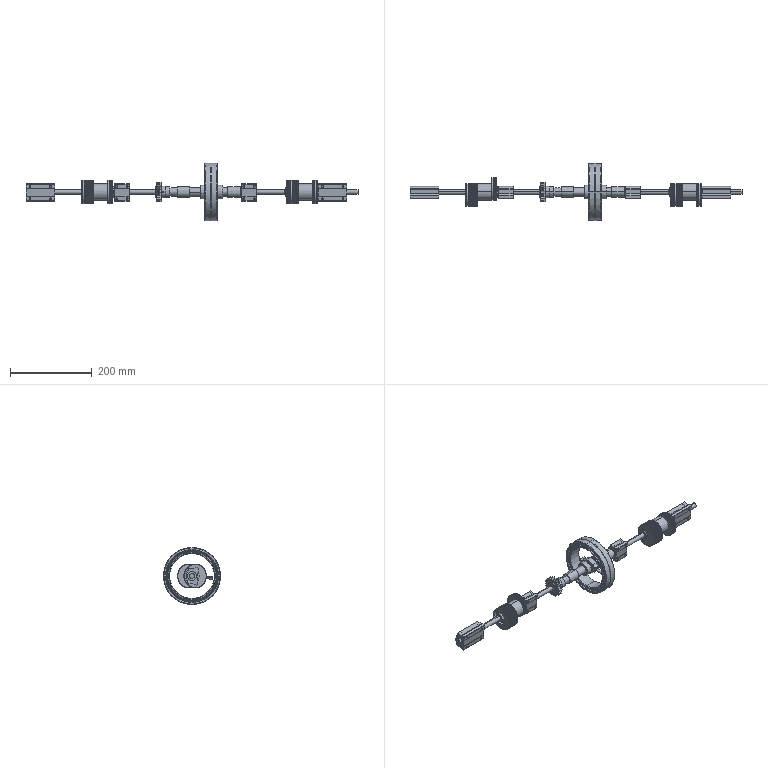Assembly | SolidWorks | mm | 26 component files | 28 solids | 3702 faces | box 814 x 140 x 140 mm | volume 749226 mm3 | plane 3023 | cylinder 492 | torus 104 | sphere 44 | cone 35 | spline 4 | commonest cylinder face diameters 5.04 x136 17.6 x48 4.3 x32 20 x28 4 x24 38.857 x23 47.978 x22 12 x18
Bill of materials:
8X8X30Coupling | 2 | AISI 1045 Steel, Cold Drawn | Plain cylindrical sleeve/spacer: solid cylinder with a single concentric smooth through-bore; length somewhat greater than outer diameter.
AxisGear(Modified) | 1 | AISI 1045 Steel, Cold Drawn | Spur gear with an integral cylindrical hub extending to one side; central round bore with a single rectangular keyway, plus a small radial hole through the hub wall.
Cam1 | 1 |  | Thin flat disc with a larger round bore containing a single rectangular keyway, plus two small through-holes placed diametrically on either side of the bore.
Cam6 | 1 |  | Thick cylindrical hub/collar with a keyed round bore and two small axial through-holes on either side of the bore.
Cam8 | 2 |  | Cylindrical hub/sleeve, roughly as long as its diameter, with a large concentric round bore having one rectangular keyway, and two small axial through-holes on opposite sides of the bore.
Cam2 | 1 |  | Thin disc with keyed round bore and two small through-holes, plus a large shallow circular recess/counterbore on one face.
Cam7 | 1 |  | Thick cylindrical hub/collar with a keyed round bore and two small axial through-holes on either side of the bore.
InnerDiameter12Slider(ExtendedVersion) | 2 | Aluminum Oxide | Elongated rectangular-profile block with a longitudinal round through-bore, side flanges carrying four mounting holes, longitudinal grooves along the faces, and a faceted/notched end profile; a recessed ring is visible at the bore end.
InnerDiameter12Slider | 2 | Aluminum Oxide | Shorter version of a prismatic block with a longitudinal round through-bore, four mounting holes in side flanges, longitudinal grooves, and a faceted/notched end profile with a recessed ring at the bore end.
IntermediateAxis | 1 | AISI 1045 Steel, Cold Drawn | Solid stepped round shaft with multiple diameter sections and a raised central collar of largest diameter.
IntermediateAxisSleeve | 1 | 5154-O, Bar (SS) | Stepped cylindrical bushing with a central large-diameter flange and smaller cylindrical bosses on each side, with a single concentric through-bore.
LongAxis(Modified) | 1 | AISI 1045 Steel, Cold Drawn | Long slender stepped shaft with a larger-diameter sleeve section and a thin flange/collar, tapering via several steps to a small-diameter tip at one end.
LongAxisUpperSleeve | 1 | 5154-O, Bar (SS) | Flanged cylindrical bushing: a short large-diameter flange joined coaxially to a longer, smaller-diameter body, with a plain through bore along the axis.
MiddleAxisUpperSleeve | 1 | 5154-O, Bar (SS) | Flanged cylindrical bushing with a through bore; the flange face has a stepped (counterbored or chamfered) bore entry and a shallow raised rim or recess near its outer edge.
needle roller bearings lm series gb | 1 |  | Thin, wide annular assembly-like body: an outer ring and an inner ring with a circumferential row of small circular elements in the annular gap between them, with a split line at mid-width on the outer surface. It looks like a thin-section rolling-element bearing.
plain parallel keys | 1 |  | Solid prismatic block with an obround (stadium-shaped) outline, i.e. a rectangle with fully rounded ends, and chamfered top and bottom edges all around. It looks like a round-ended parallel key.
ShortAxis(Modified) | 1 | AISI 1045 Steel, Cold Drawn | Long slender stepped shaft: a short reduced-diameter pin at one end, a long main shaft, a central larger-diameter collar section with a thin flange/rim at one end, then the shaft continues to a plain end.
Sleeve(Modified) | 1 | Plain Carbon Steel | Split clamp body: a ring with a large circular bore, a radial slit from the bore out to two parallel clamping tabs, a small cross hole through the tabs, and a cylindrical rod sticking out radially from the side opposite the slit.
taper keys for general use gb | 2 |  | Solid obround (stadium-outline) block with chamfered perimeter edges, longer and slimmer than the similar block unnamed part. It looks like a round-ended parallel key.
thrust ball bearings gb | 2 |  | Thrust-bearing-like stack: two flat annular washers with central bores, separated by a single circular row of spherical balls.
Mates:
1. concentric | LongAxis(Modified)-1 face at (52.062, 28.116, 349) dir (0, -1, 0) r 1.5 | plain parallel keys-1 face at (60.062, 18.116, 349) dir (0, 1, 0) r 1.5
2. concentric | LongAxis(Modified)-1 face at (65.062, 28.116, 349) dir (0, -1, 0) r 1.5 | plain parallel keys-1 face at (65.062, 18.116, 349) dir (0, 1, 0) r 1.5
3. coincident | LongAxis(Modified)-1 face at (65.062, 18.116, 349) dir (0, 1, 0) | plain parallel keys-1 face at (60.062, 18.116, 349) dir (0, -1, 0)
4. concentric | LongAxis(Modified)-1 face at (-73.938, 31.616, 349) dir (0, -1, 0) r 3 | taper keys for general use gb-1 face at (-73.938, 21.616, 349) dir (0, 1, 0) r 1
5. coincident | LongAxis(Modified)-1 face at (-73.938, 21.616, 349) dir (0, 1, 0) | taper keys for general use gb-1 face at (-77.938, 21.616, 349) dir (0, -1, 0)
6. coincident | LongAxis(Modified)-1 face at (-144.532, 31.616, 352) dir (0, 0, -1) | taper keys for general use gb-1 face at (-77.938, 21.616, 350) dir (0, 0, 1)
7. concentric | LongAxis(Modified)-1 face at (-233.938, 15.116, 349) dir (-1, 0, 0) r 4.5 | AxisGear(Modified)-1 face at (47.062, 15.116, 349) dir (1, 0, 0) r 4.5
8. coincident | plain parallel keys-1 face at (60.062, 18.116, 350.5) dir (0, 0, 1) | AxisGear(Modified)-1 face at (47.062, 21.116, 350.5) dir (0, 0, -1)
9. coincident | LongAxis(Modified)-1 face at (47.062, 21.116, 349) dir (1, 0, 0) | AxisGear(Modified)-1 face at (47.062, 15.116, 349) dir (-1, 0, 0)
10. concentric | LongAxis(Modified)-1 face at (-233.938, 15.116, 349) dir (-1, 0, 0) r 4 | LongAxisUpperSleeve-1 face at (-2.883, 15.116, 349) dir (-1, 0, 0) r 4
11. coincident | AxisGear(Modified)-1 face at (72.062, 15.116, 349) dir (1, 0, 0) | LongAxisUpperSleeve-1 face at (72.062, 28.116, 349) dir (-1, 0, 0)
12. concentric | LongAxis(Modified)-1 face at (-233.938, 15.116, 349) dir (-1, 0, 0) r 4 | 8X8X30Coupling-1 face at (100.062, 15.116, 349) dir (1, 0, 0) r 4
13. coincident | LongAxisUpperSleeve-1 face at (100.062, 25.116, 349) dir (1, 0, 0) | 8X8X30Coupling-1 face at (100.062, 15.116, 349) dir (-1, 0, 0)
14. concentric | IntermediateAxis-1 face at (-31.245, 15.116, 349) dir (-1, 0, 0) r 4 | 8X8X30Coupling-1 face at (100.062, 15.116, 349) dir (1, 0, 0) r 4
15. coincident | IntermediateAxis-1 face at (130.062, 19.116, 349) dir (-1, 0, 0) | 8X8X30Coupling-1 face at (130.062, 15.116, 349) dir (1, 0, 0)
16. concentric | IntermediateAxis-1 face at (-31.245, 15.116, 349) dir (-1, 0, 0) r 6 | needle roller bearings lm series gb-1 face at (167.562, 15.116, 349) dir (-1, 0, 0) r 55
17. coincident | IntermediateAxis-1 face at (176.062, 23.116, 349) dir (1, 0, 0) | needle roller bearings lm series gb-1 face at (167.562, 15.116, 349) dir (-1, 0, 0)
18. concentric | IntermediateAxis-1 face at (-31.245, 15.116, 349) dir (-1, 0, 0) r 5 | MiddleAxisUpperSleeve-1 face at (242.008, 15.116, 349) dir (1, 0, 0) r 5
19. concentric | IntermediateAxis-1 face at (-31.245, 15.116, 349) dir (-1, 0, 0) r 8 | thrust ball bearings gb-1 face at (166.688, 15.116, 349) dir (-1, 0, 0) r 5
20. concentric | needle roller bearings lm series gb-1 face at (167.562, 15.116, 349) dir (-1, 0, 0) r 70 | Sleeve(Modified)-1 face at (176.062, 15.116, 349) dir (1, 0, 0) r 12
21. coincident | needle roller bearings lm series gb-1 face at (197.562, 15.116, 349) dir (1, 0, 0) | Sleeve(Modified)-1 face at (189.062, 15.116, 349) dir (1, 0, 0)
22. coincident | thrust ball bearings gb-1 face at (176.062, 20.116, 349) dir (1, 0, 0) | Sleeve(Modified)-1 face at (176.062, 15.116, 349) dir (-1, 0, 0)
23. coincident | MiddleAxisUpperSleeve-1 face at (167.062, 18.792, 334.458) dir (1, 0, 0) | thrust ball bearings gb-1 face at (167.062, 20.116, 349) dir (-1, 0, 0)
24. concentric | IntermediateAxis-1 face at (-31.245, 15.116, 349) dir (-1, 0, 0) r 5 | thrust ball bearings gb-2 face at (188.688, 15.116, 349) dir (-1, 0, 0) r 5
25. coincident | Sleeve(Modified)-1 face at (189.062, 15.116, 349) dir (1, 0, 0) | thrust ball bearings gb-2 face at (189.062, 20.116, 349) dir (-1, 0, 0)
26. concentric | IntermediateAxis-1 face at (-31.245, 15.116, 349) dir (-1, 0, 0) r 5 | IntermediateAxisSleeve-1 face at (127.408, 15.116, 349) dir (-1, 0, 0) r 5
27. coincident | IntermediateAxisSleeve-1 face at (198.062, 23.116, 349) dir (-1, 0, 0) | thrust ball bearings gb-2 face at (198.062, 20.116, 349) dir (1, 0, 0)
28. concentric | IntermediateAxis-1 face at (-31.245, 15.116, 349) dir (-1, 0, 0) r 4 | 8X8X30Coupling-2 face at (224.062, 15.116, 349) dir (1, 0, 0) r 4
29. coincident | IntermediateAxisSleeve-1 face at (224.062, 25.116, 349) dir (1, 0, 0) | 8X8X30Coupling-2 face at (224.062, 15.116, 349) dir (-1, 0, 0)
30. concentric | 8X8X30Coupling-2 face at (224.062, 15.116, 349) dir (1, 0, 0) r 4 | ShortAxis(Modified)-1 face at (543.062, 15.116, 349) dir (1, 0, 0) r 4
31. coincident | 8X8X30Coupling-2 face at (254.062, 15.116, 349) dir (1, 0, 0) | ShortAxis(Modified)-1 face at (254.062, 21.116, 349) dir (-1, 0, 0)
32. concentric | ShortAxis(Modified)-1 face at (383.062, 31.616, 349) dir (0, -1, 0) r 3 | taper keys for general use gb-2 face at (383.062, 21.616, 349) dir (0, 1, 0) r 1
33. coincident | ShortAxis(Modified)-1 face at (443.062, 21.116, 349) dir (1, 0, 0) | taper keys for general use gb-2 face at (443.062, 90.587, 346) dir (1, 0, 0)
34. coincident | ShortAxis(Modified)-1 face at (383.062, 21.616, 349) dir (0, 1, 0) | taper keys for general use gb-2 face at (387.062, 21.616, 349) dir (0, -1, 0)
35. concentric | LongAxis(Modified)-1 face at (-233.938, 15.116, 349) dir (-1, 0, 0) r 6 | InnerDiameter12Slider(ExtendedVersion)-1 face at (-200.938, 15.116, 349) dir (-1, 0, 0) r 6
36. concentric | LongAxis(Modified)-1 face at (-233.938, 15.116, 349) dir (-1, 0, 0) r 6 | InnerDiameter12Slider-1 face at (-17.938, 15.116, 349) dir (-1, 0, 0) r 6
37. concentric | ShortAxis(Modified)-1 face at (543.062, 15.116, 349) dir (1, 0, 0) r 6 | InnerDiameter12Slider-2 face at (294.062, 15.116, 349) dir (-1, 0, 0) r 6
38. concentric | ShortAxis(Modified)-1 face at (543.062, 15.116, 349) dir (1, 0, 0) r 6 | InnerDiameter12Slider(ExtendedVersion)-2 face at (516.062, 15.116, 349) dir (-1, 0, 0) r 6
39. coincident | InnerDiameter12Slider(ExtendedVersion)-1 face at (-200.938, -1.722, 367.438) dir (0, -0.9954, -0.09551) | InnerDiameter12Slider-1 face at (-17.938, -1.722, 367.438) dir (0, -0.9954, -0.09551)
40. coincident | InnerDiameter12Slider(ExtendedVersion)-2 face at (516.062, -1.722, 367.438) dir (0, -0.9954, -0.09551) | InnerDiameter12Slider-2 face at (294.062, -1.722, 367.438) dir (0, -0.9954, -0.09551)
41. coincident | InnerDiameter12Slider-1 face at (-17.938, -1.722, 367.438) dir (0, -0.9954, -0.09551) | InnerDiameter12Slider-2 face at (294.062, -1.722, 367.438) dir (0, -0.9954, -0.09551)
42. distance | InnerDiameter12Slider(ExtendedVersion)-1 face at (-200.938, 15.116, 349) dir (1, 0, 0) | InnerDiameter12Slider-1 face at (-53.938, 15.116, 349) dir (-1, 0, 0)
43. distance | InnerDiameter12Slider-2 face at (294.062, 15.116, 349) dir (1, 0, 0) | InnerDiameter12Slider(ExtendedVersion)-2 face at (446.062, 15.116, 349) dir (-1, 0, 0)
44. distance | InnerDiameter12Slider-1 face at (-53.938, 15.116, 349) dir (-1, 0, 0) | LongAxis(Modified)-1 face at (-55.938, 28.116, 349) dir (1, 0, 0)
45. distance | InnerDiameter12Slider(ExtendedVersion)-2 face at (446.062, 15.116, 349) dir (-1, 0, 0) | ShortAxis(Modified)-1 face at (443.062, 21.116, 349) dir (1, 0, 0)
46. parallel | Sleeve(Modified)-1 face at (176.062, -5.461, 354.058) dir (0, -0.9954, -0.09551) | InnerDiameter12Slider-1 face at (-17.938, -1.722, 367.438) dir (0, -0.9954, -0.09551)
47. parallel | Sleeve(Modified)-1 face at (176.062, -5.461, 354.058) dir (0, -0.9954, -0.09551) | InnerDiameter12Slider-2 face at (294.062, -1.722, 367.438) dir (0, -0.9954, -0.09551)
48. parallel | InnerDiameter12Slider(ExtendedVersion)-1 face at (-200.938, -1.722, 367.438) dir (0, -0.9954, -0.09551) | InnerDiameter12Slider-1 face at (-17.938, -1.722, 367.438) dir (0, -0.9954, -0.09551)
49. coincident | LongAxis(Modified)-1 face at (-58.938, 25.116, 349) dir (-1, 0, 0) | CamGroup3-1/Cam1-1 face at (-58.938, 131.977, 452.927) dir (1, 0, 0)
50. concentric | LongAxis(Modified)-1 face at (-233.938, 15.116, 349) dir (-1, 0, 0) r 10 | CamGroup3-1/Cam6-1 face at (-124.938, 15.116, 349) dir (-1, 0, 0) r 18
51. parallel | taper keys for general use gb-1 face at (-73.938, 21.616, 348) dir (0, 0, -1) | CamGroup3-1/Cam6-1 face at (-133.938, 27.9, 346) dir (0, 0, 1)
52. coincident | ShortAxis(Modified)-1 face at (368.062, 25.116, 349) dir (1, 0, 0) | CamGroup4-1/Cam7-1 face at (368.062, -101.746, 452.927) dir (-1, 0, 0)
53. concentric | ShortAxis(Modified)-1 face at (543.062, 15.116, 349) dir (1, 0, 0) r 10 | CamGroup4-1/Cam2-1 face at (434.062, 15.116, 349) dir (1, 0, 0) r 18
54. parallel | taper keys for general use gb-2 face at (383.062, 21.616, 350) dir (0, 0, 1) | CamGroup4-1/Cam2-1 face at (443.062, 27.905, 352) dir (0, 0, -1)
55. coincident | Cam1-1 face at (-101.594, -111.592, 63.075) dir (0, 0, 1) | Cam8-1 face at (2.333, 5.272, 63.075) dir (0, 0, -1)
56. concentric | Cam1-1 face at (-13.667, 5.27, 63.075) dir (0, 0, -1) r 2 | Cam8-1 face at (-13.667, 5.27, 98.075) dir (0, 0, -1) r 2
57. concentric | Cam1-1 face at (18.333, 5.27, 63.075) dir (0, 0, -1) r 2 | Cam8-1 face at (18.333, 5.27, 98.075) dir (0, 0, -1) r 2
58. coincident | Cam8-1 face at (2.333, 5.272, 98.075) dir (0, 0, 1) | Cam6-1 face at (106.261, 122.132, 98.075) dir (0, 0, -1)
59. concentric | Cam8-1 face at (-13.667, 5.27, 98.075) dir (0, 0, -1) r 2 | Cam6-1 face at (-13.667, 5.27, 127.075) dir (0, 0, -1) r 2
60. concentric | Cam8-1 face at (18.333, 5.27, 98.075) dir (0, 0, -1) r 2 | Cam6-1 face at (18.333, 5.27, 127.075) dir (0, 0, -1) r 2
61. coincident | Cam2-1 face at (-100.985, -113.925, 52.075) dir (0, 0, -1) | Cam8-1 face at (2.942, 2.932, 52.075) dir (0, 0, 1)
62. concentric | Cam2-1 face at (-13.058, 2.935, 63.075) dir (0, 0, -1) r 2 | Cam8-1 face at (-13.058, 2.935, 52.075) dir (0, 0, -1) r 2
63. concentric | Cam2-1 face at (18.942, 2.935, 63.075) dir (0, 0, -1) r 2 | Cam8-1 face at (18.942, 2.935, 52.075) dir (0, 0, -1) r 2
64. coincident | Cam8-1 face at (2.942, 2.932, 17.075) dir (0, 0, -1) | Cam7-1 face at (-100.985, -113.927, 17.075) dir (0, 0, 1)
65. concentric | Cam8-1 face at (-13.058, 2.935, 52.075) dir (0, 0, -1) r 2 | Cam7-1 face at (-13.058, 2.935, 17.075) dir (0, 0, -1) r 2
66. concentric | Cam8-1 face at (18.942, 2.935, 52.075) dir (0, 0, -1) r 2 | Cam7-1 face at (18.942, 2.935, 17.075) dir (0, 0, -1) r 2